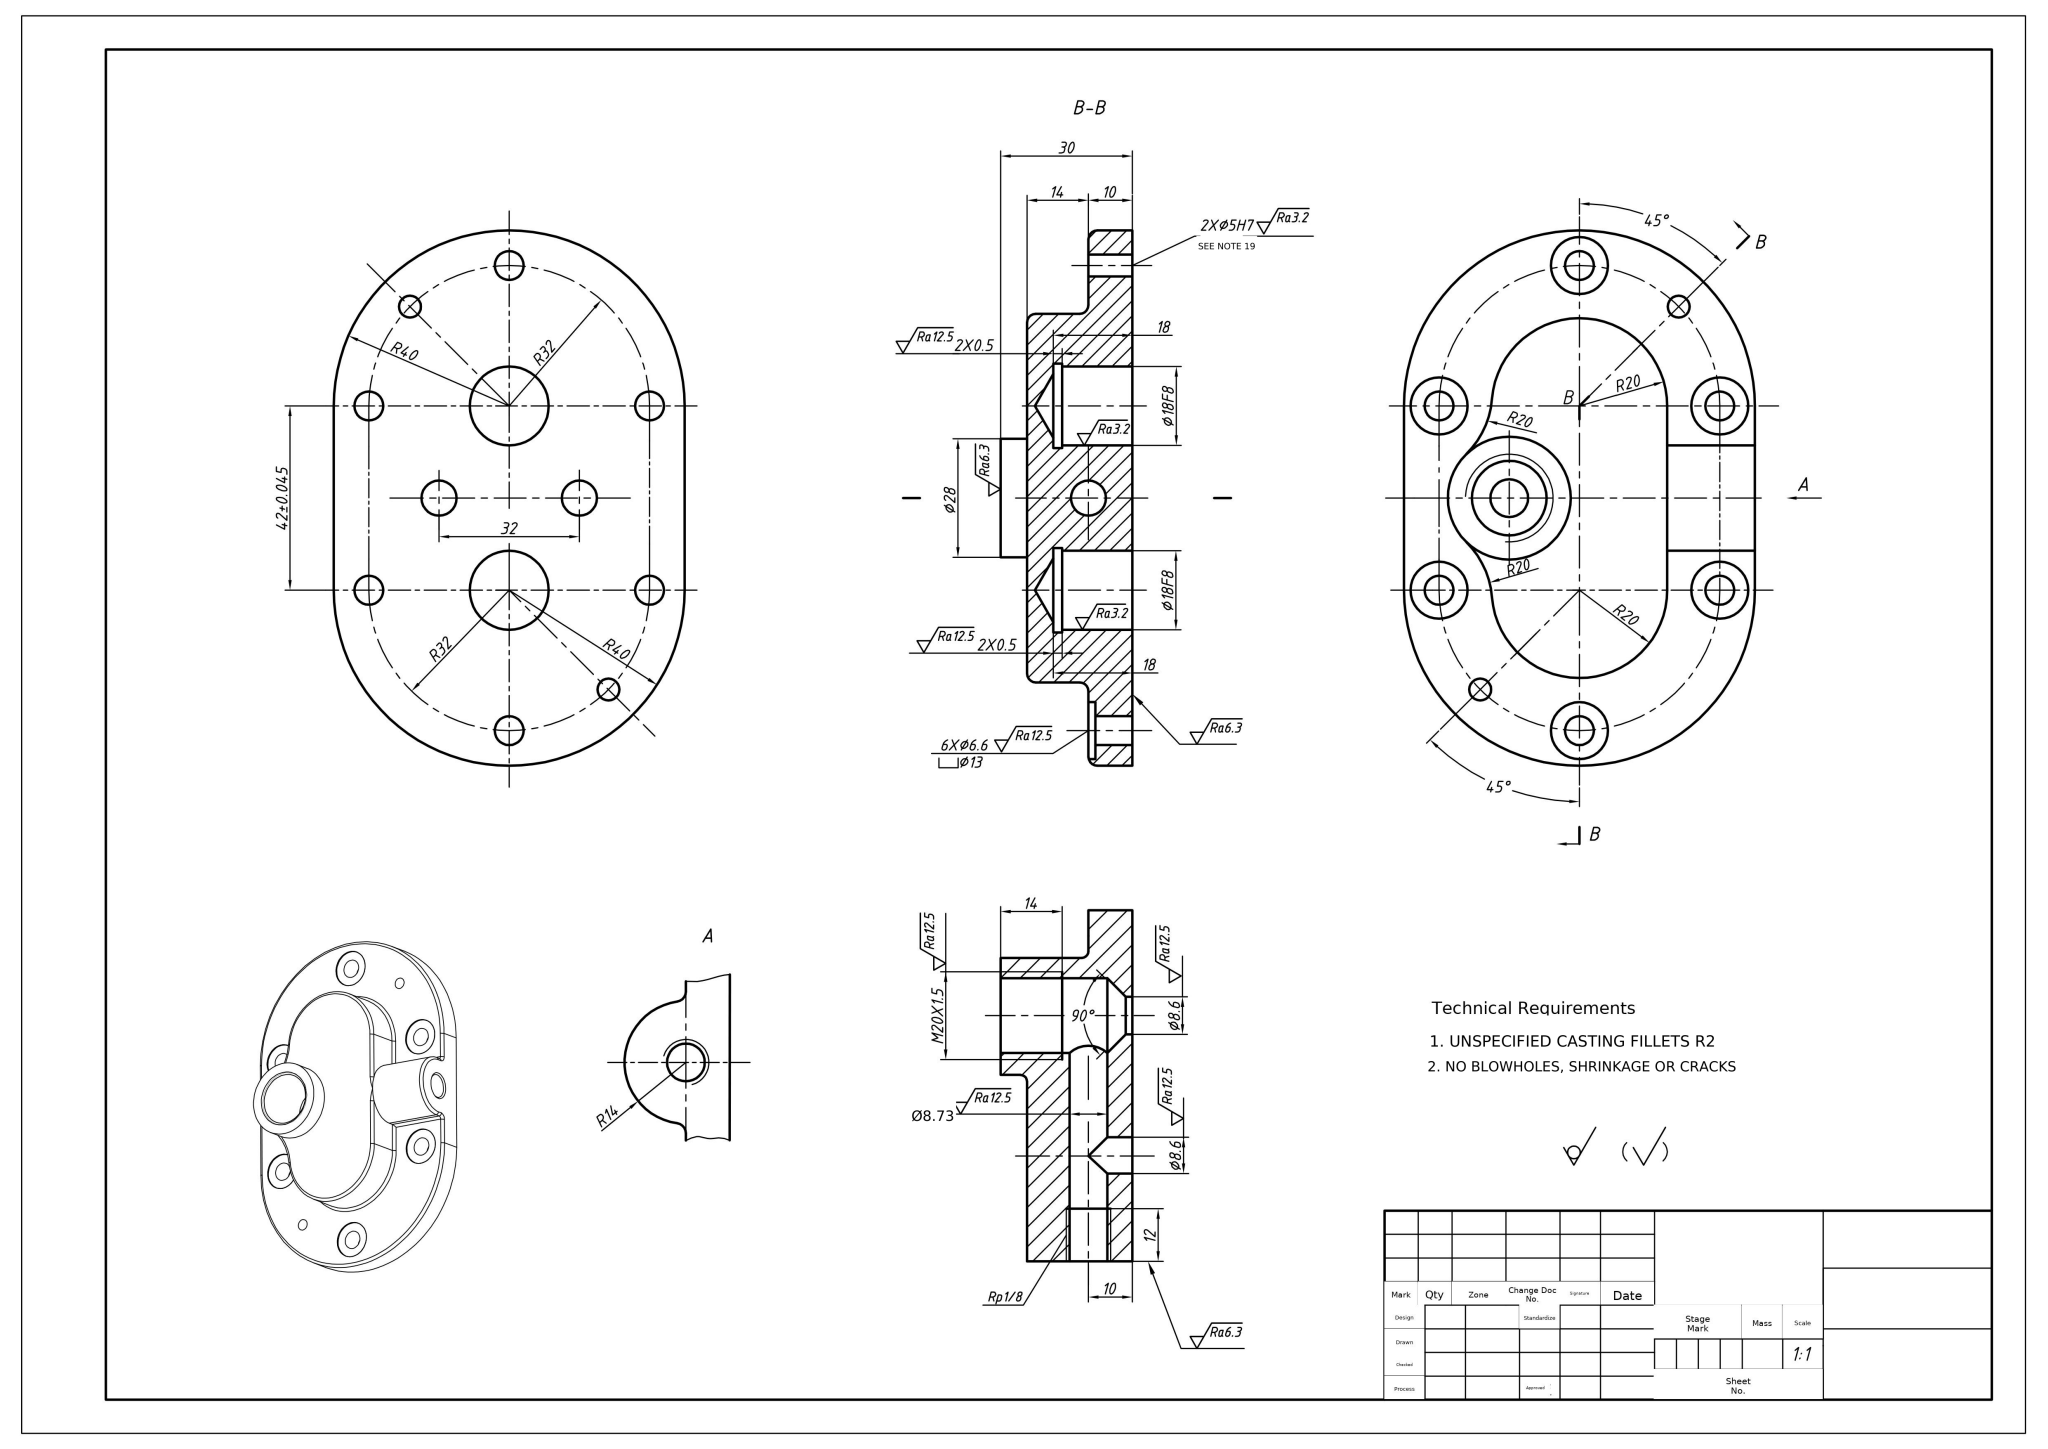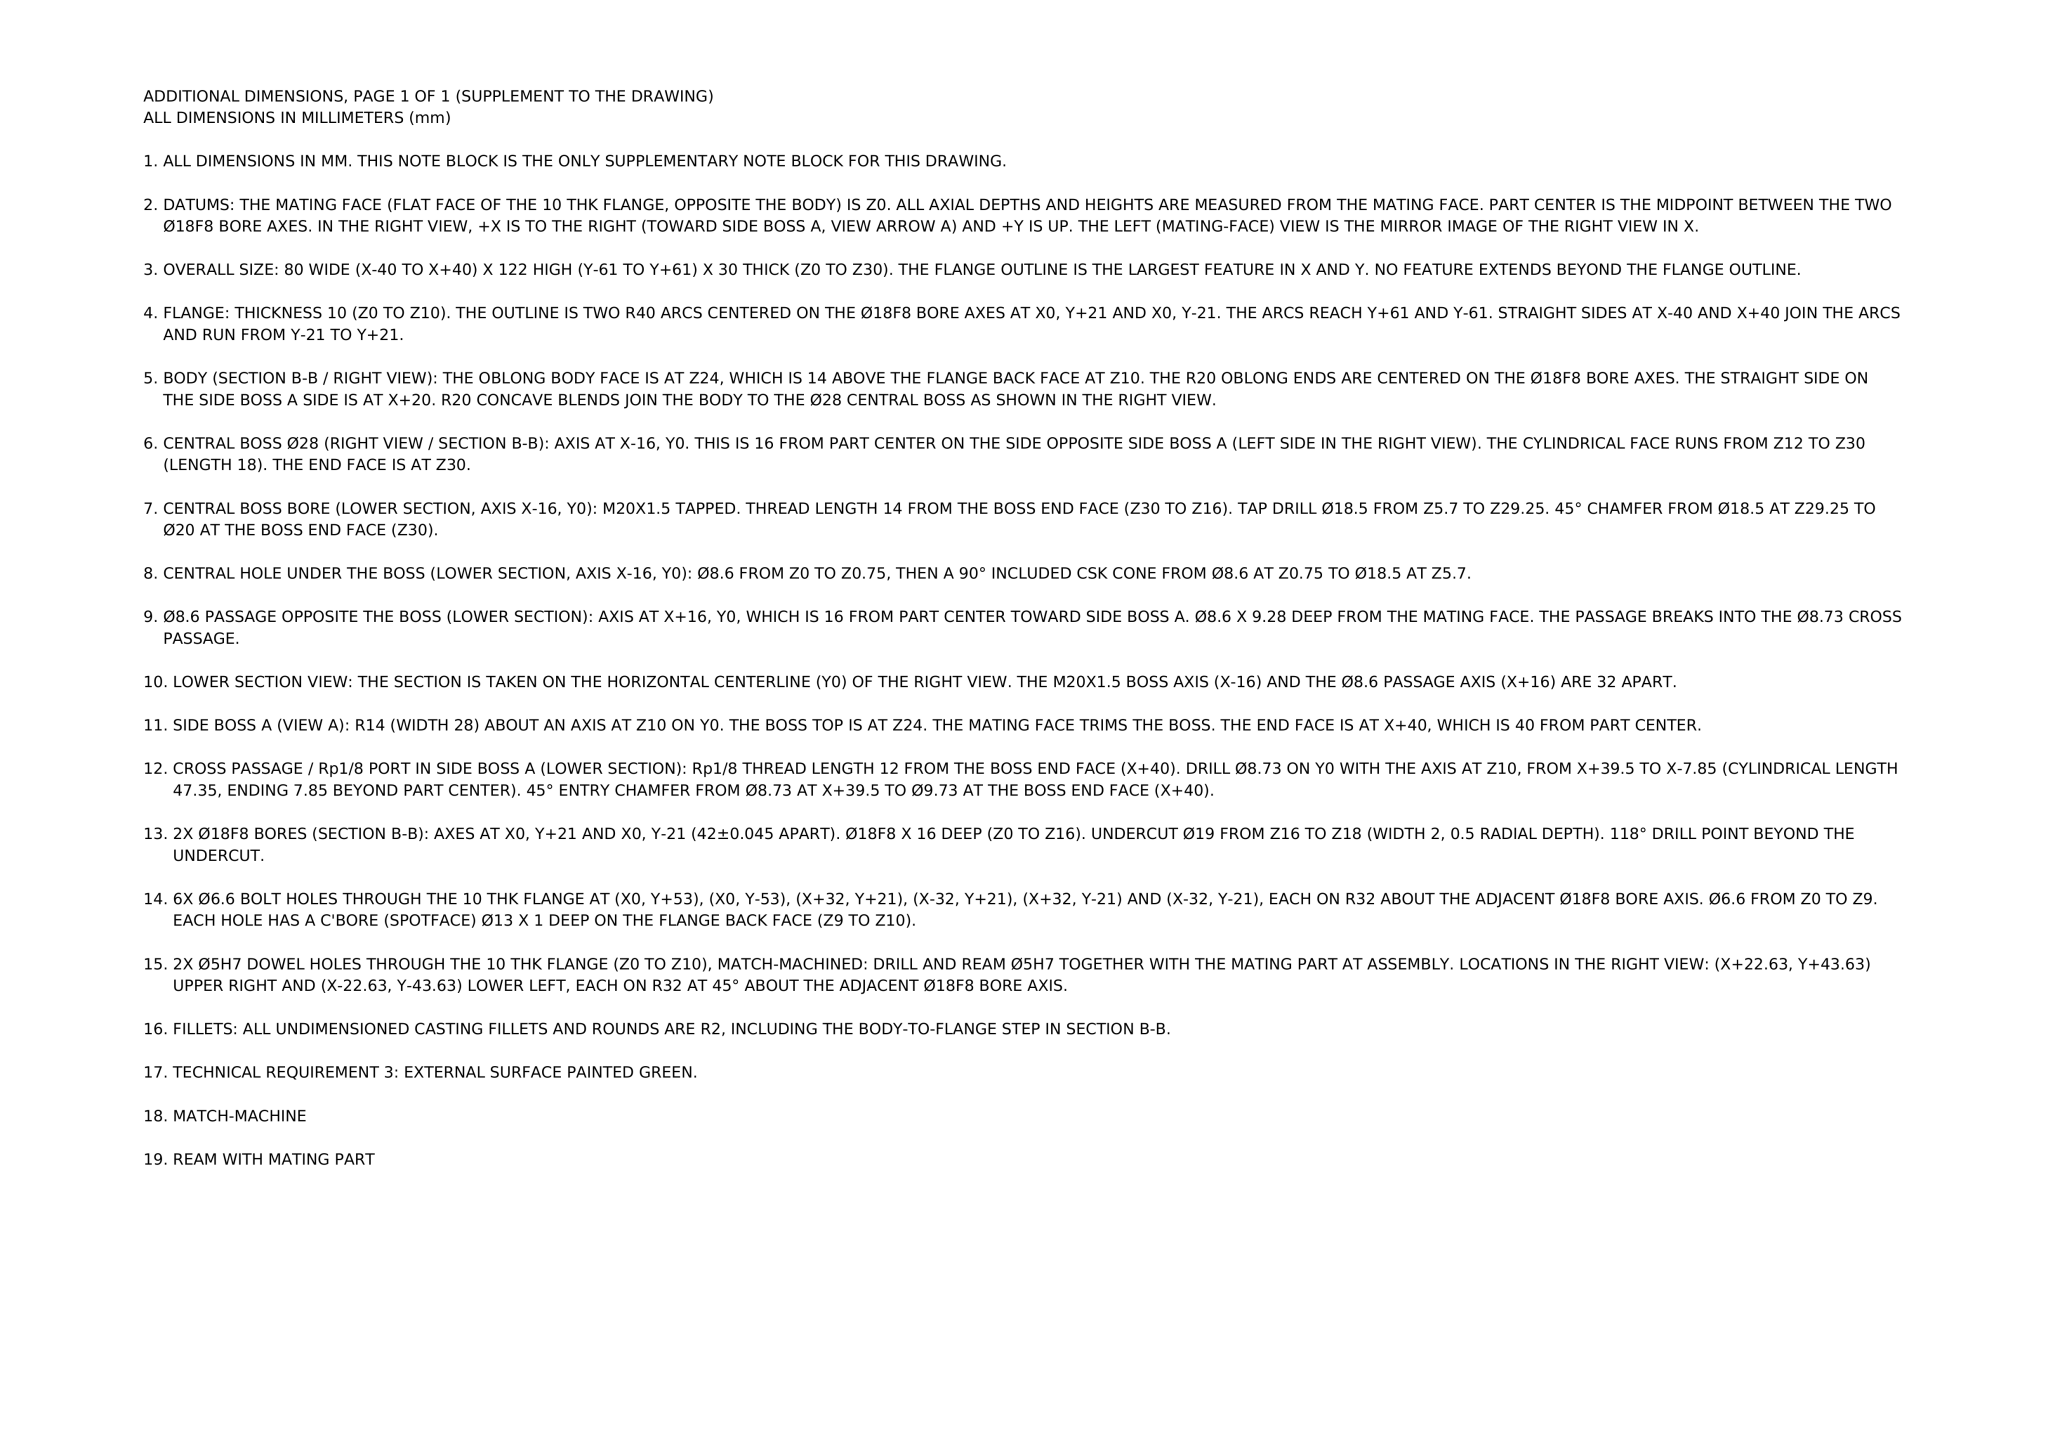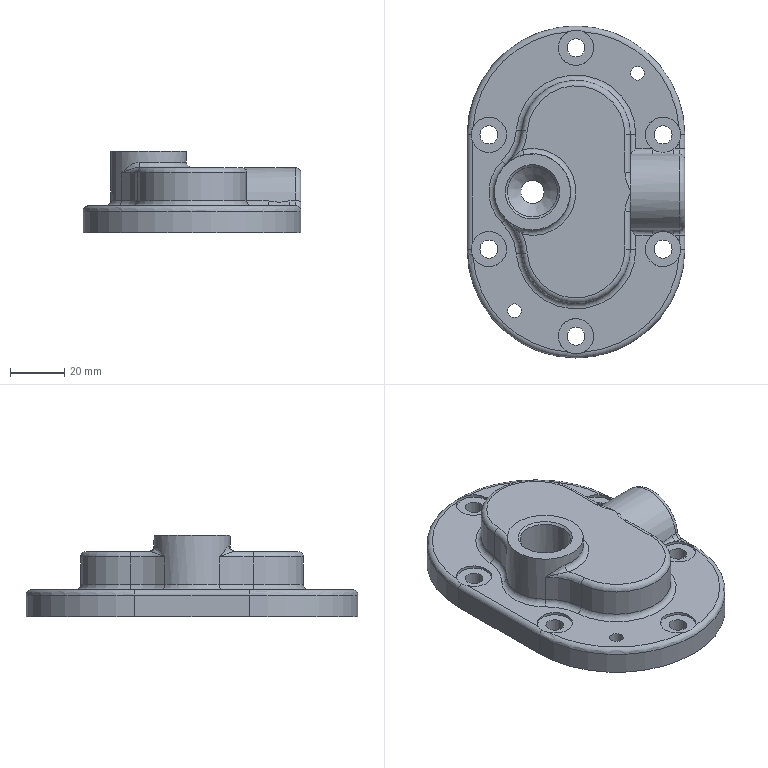Part | NX | mm | 1 solid | 87 faces | box 80 x 122 x 30 mm | volume 113986 mm3 | cylinder 41 | plane 20 | torus 15 | spline 6 | cone 5 | commonest cylinder face diameters 4 x11 6.6 x6 13 x6 40 x4 18 x2 80 x2 28 x2 5 x2